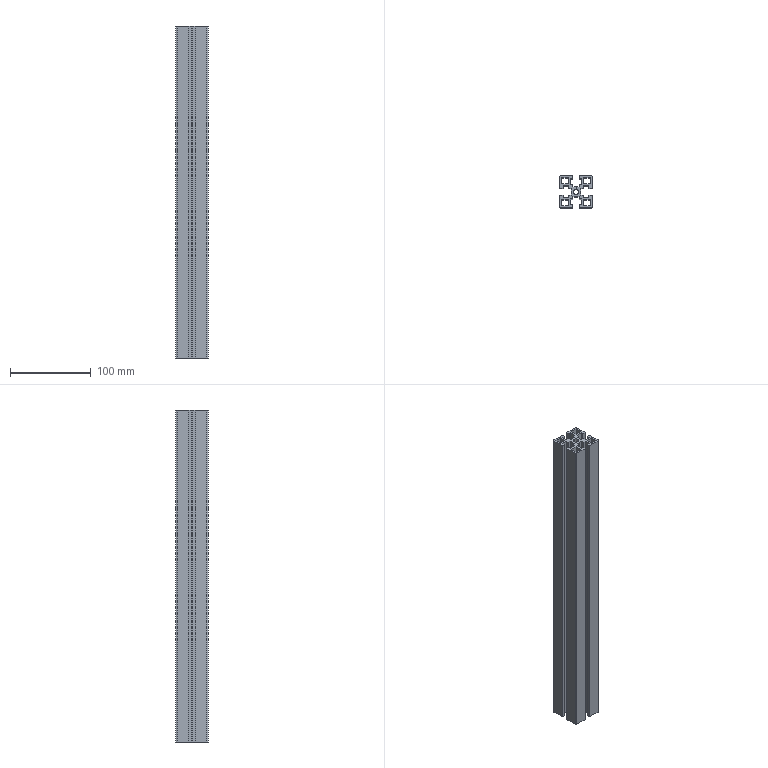Component | SolidWorks | 4040-410AluminumProfile-1 | 1 solid | 88 faces | box 40 x 40 x 410 mm | volume 279554 mm3 | plane 82 | cylinder 6 | commonest cylinder face diameters 3 x4 6.8 x2 | material A6061
build123d program:
from build123d import *

# Parameters (mm, degrees)
SKETCH11_R                    = 3.4
SKETCH11_W                    = 7.85
SKETCH11_H                    = 7.85
ALUMINUM_PROFILE_4040_1_DEPTH = 410


with BuildPart() as part:
    # Sketch11 → Aluminum Profile 4040_1 (new body)
    with BuildSketch(Plane(origin=(0, 0, 0), x_dir=(0, 0, -1), z_dir=(1, 0, 0))):
        with BuildLine():
            Line((18.5, 20), (4.15, 20))
            Line((4.15, 20), (4.15, 16))
            Line((4.15, 16), (7.15, 16))
            Line((7.15, 16), (7.15, 9))
            Line((7.15, 9), (4.15, 9))
            Line((4.15, 9), (4.15, 6))
            Line((4.15, 6), (0.52, 6))
            Line((0.52, 6), (0, 5.7))
            Line((0, 5.7), (-0.519, 6))
            Line((-0.519, 6), (-4.15, 6))
            Line((-4.15, 6), (-4.15, 9))
            Line((-4.15, 9), (-7.15, 9))
            Line((-7.15, 9), (-7.15, 16))
            Line((-7.15, 16), (-4.15, 16))
            Line((-4.15, 16), (-4.15, 20))
            Line((-4.15, 20), (-18.5, 20))
            ThreePointArc((-18.5, 20), (-19.561, 19.561), (-20, 18.5))
            Line((-20, 18.5), (-20, 4.15))
            Line((-20, 4.15), (-16, 4.15))
            Line((-16, 4.15), (-16, 7.15))
            Line((-16, 7.15), (-9, 7.15))
            Line((-9, 7.15), (-9, 4.15))
            Line((-9, 4.15), (-6, 4.15))
            Line((-6, 4.15), (-6, 0.52))
            Line((-6, 0.52), (-5.7, 0))
            Line((-5.7, 0), (-6, -0.519))
            Line((-6, -0.519), (-6, -4.15))
            Line((-6, -4.15), (-9, -4.15))
            Line((-9, -4.15), (-9, -7.15))
            Line((-9, -7.15), (-16, -7.15))
            Line((-16, -7.15), (-16, -4.15))
            Line((-16, -4.15), (-20, -4.15))
            Line((-20, -4.15), (-20, -18.5))
            ThreePointArc((-20, -18.5), (-19.561, -19.561), (-18.5, -20))
            Line((-18.5, -20), (-4.15, -20))
            Line((-4.15, -20), (-4.15, -16))
            Line((-4.15, -16), (-7.15, -16))
            Line((-7.15, -16), (-7.15, -9))
            Line((-7.15, -9), (-4.15, -9))
            Line((-4.15, -9), (-4.15, -6))
            Line((-4.15, -6), (-0.519, -6))
            Line((-0.519, -6), (0, -5.7))
            Line((0, -5.7), (0.52, -6))
            Line((0.52, -6), (4.15, -6))
            Line((4.15, -6), (4.15, -9))
            Line((4.15, -9), (7.15, -9))
            Line((7.15, -9), (7.15, -16))
            Line((7.15, -16), (4.15, -16))
            Line((4.15, -16), (4.15, -20))
            Line((4.15, -20), (18.5, -20))
            ThreePointArc((18.5, -20), (19.561, -19.561), (20, -18.5))
            Line((20, -18.5), (20, -4.15))
            Line((20, -4.15), (16, -4.15))
            Line((16, -4.15), (16, -7.15))
            Line((16, -7.15), (9, -7.15))
            Line((9, -7.15), (9, -4.15))
            Line((9, -4.15), (6, -4.15))
            Line((6, -4.15), (6, -0.519))
            Line((6, -0.519), (5.7, 0))
            Line((5.7, 0), (6, 0.52))
            Line((6, 0.52), (6, 4.15))
            Line((6, 4.15), (9, 4.15))
            Line((9, 4.15), (9, 7.15))
            Line((9, 7.15), (16, 7.15))
            Line((16, 7.15), (16, 4.15))
            Line((16, 4.15), (20, 4.15))
            Line((20, 4.15), (20, 18.5))
            ThreePointArc((20, 18.5), (19.561, 19.561), (18.5, 20))
        make_face()
        Circle(SKETCH11_R, mode=Mode.SUBTRACT)
        with Locations((-13.575, 13.575)):
            Rectangle(SKETCH11_W, SKETCH11_H, mode=Mode.SUBTRACT)
        with Locations((-13.575, -13.575)):
            Rectangle(SKETCH11_W, SKETCH11_H, mode=Mode.SUBTRACT)
        with Locations((13.575, 13.575)):
            Rectangle(SKETCH11_W, SKETCH11_H, mode=Mode.SUBTRACT)
        with Locations((13.575, -13.575)):
            Rectangle(SKETCH11_W, SKETCH11_H, mode=Mode.SUBTRACT)
    extrude(amount=ALUMINUM_PROFILE_4040_1_DEPTH)


solid = part.part

# Placed as in the assembly
solid = solid.moved(Location((-58.503, 105.215, 410.05), (0, 90, 0)))